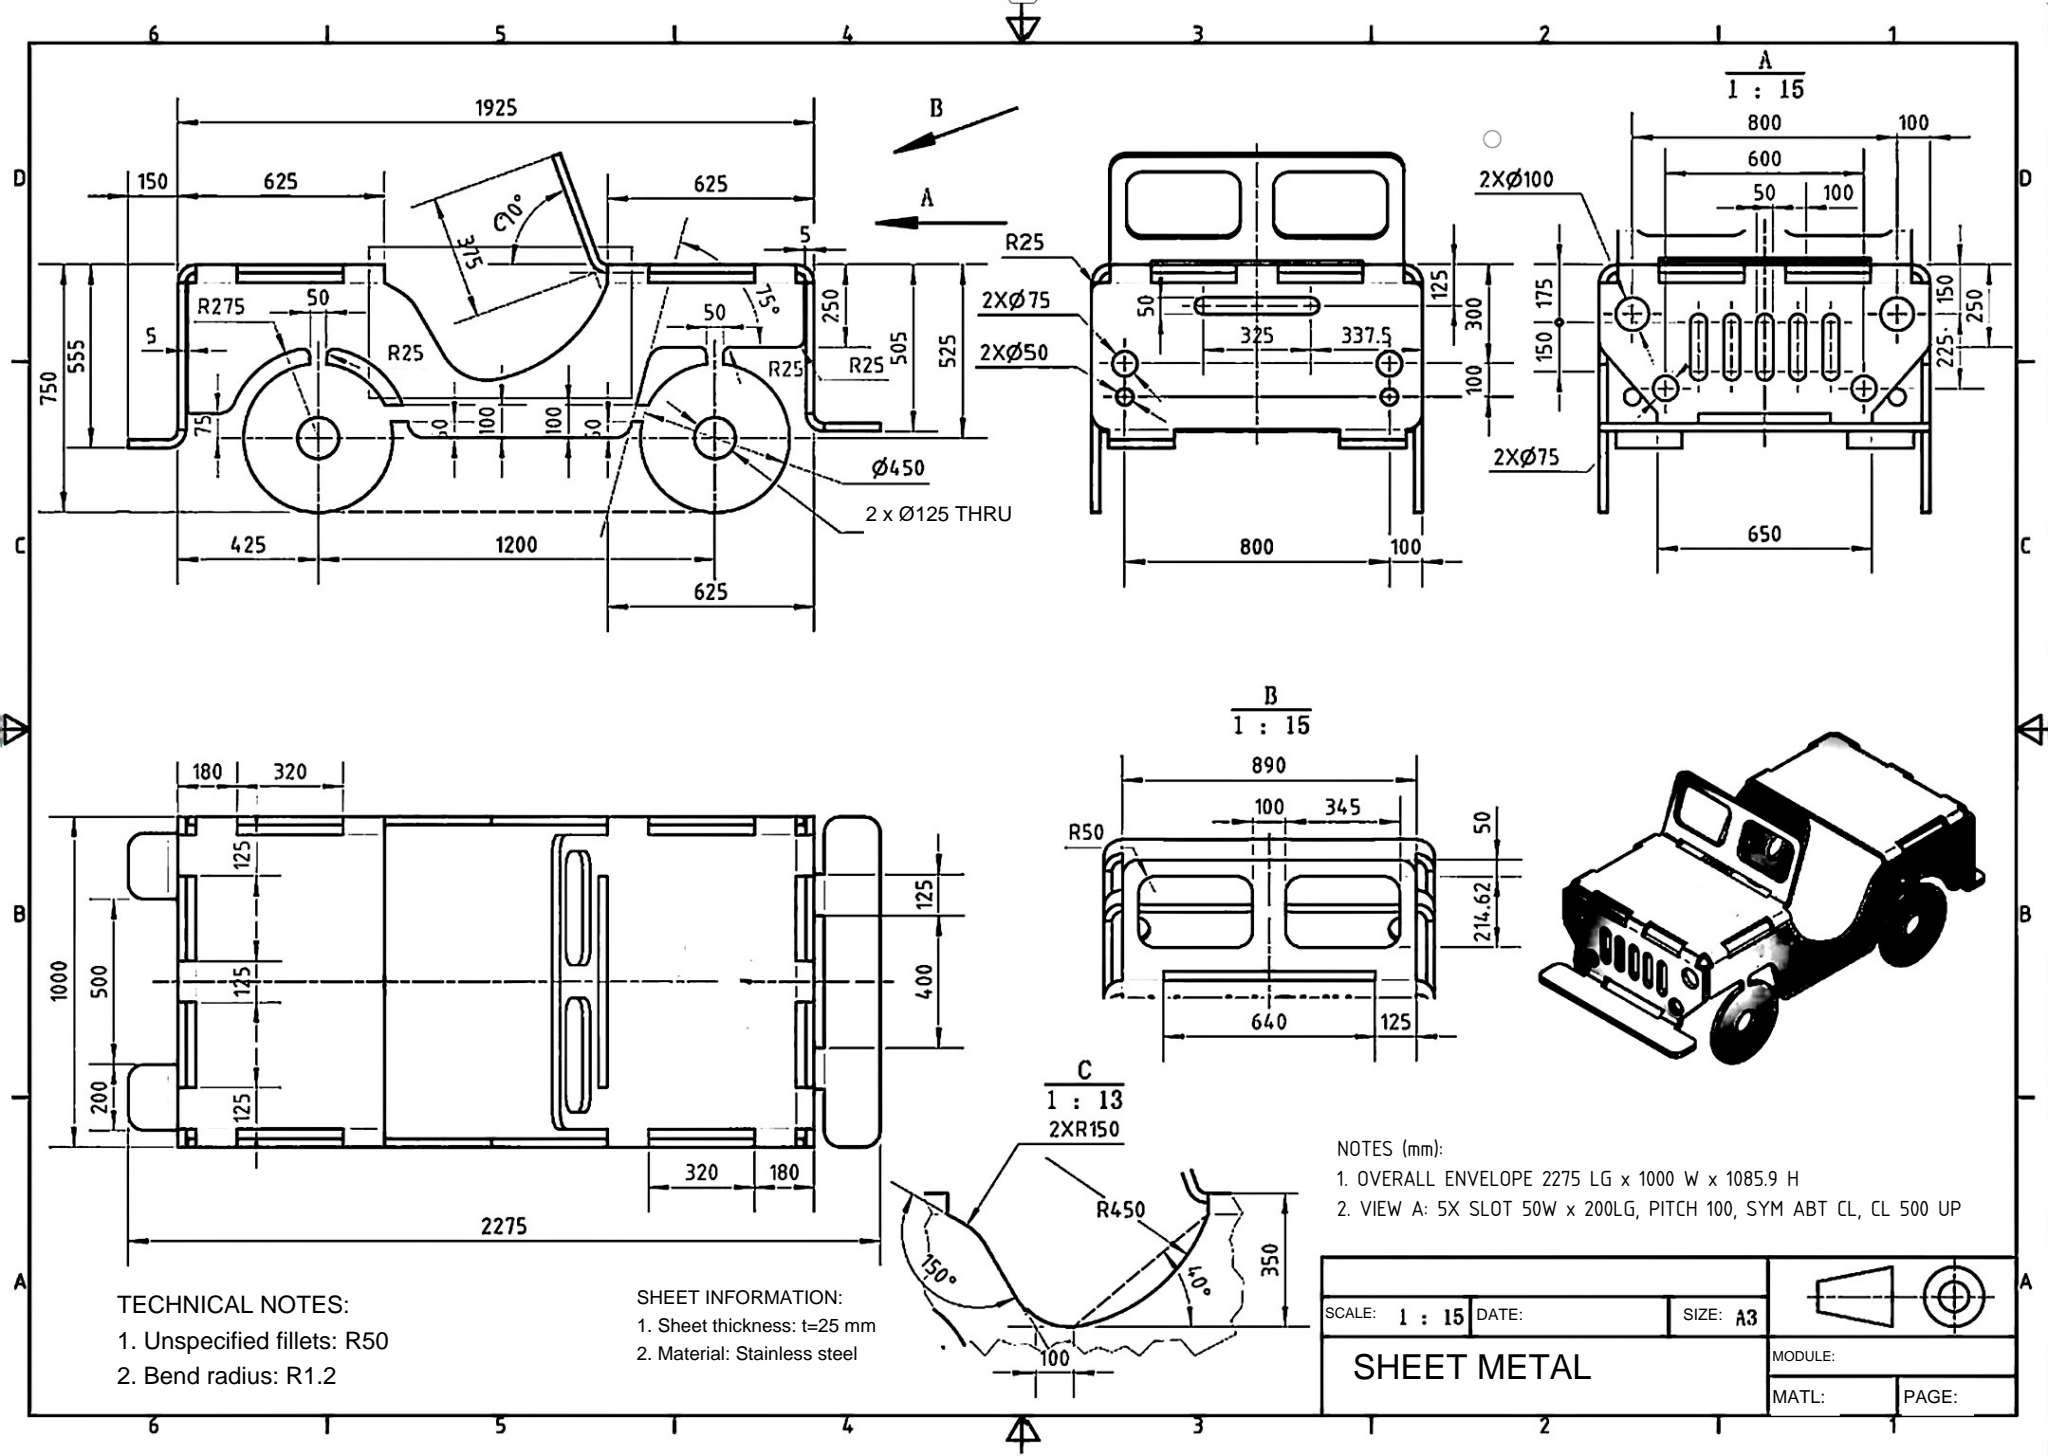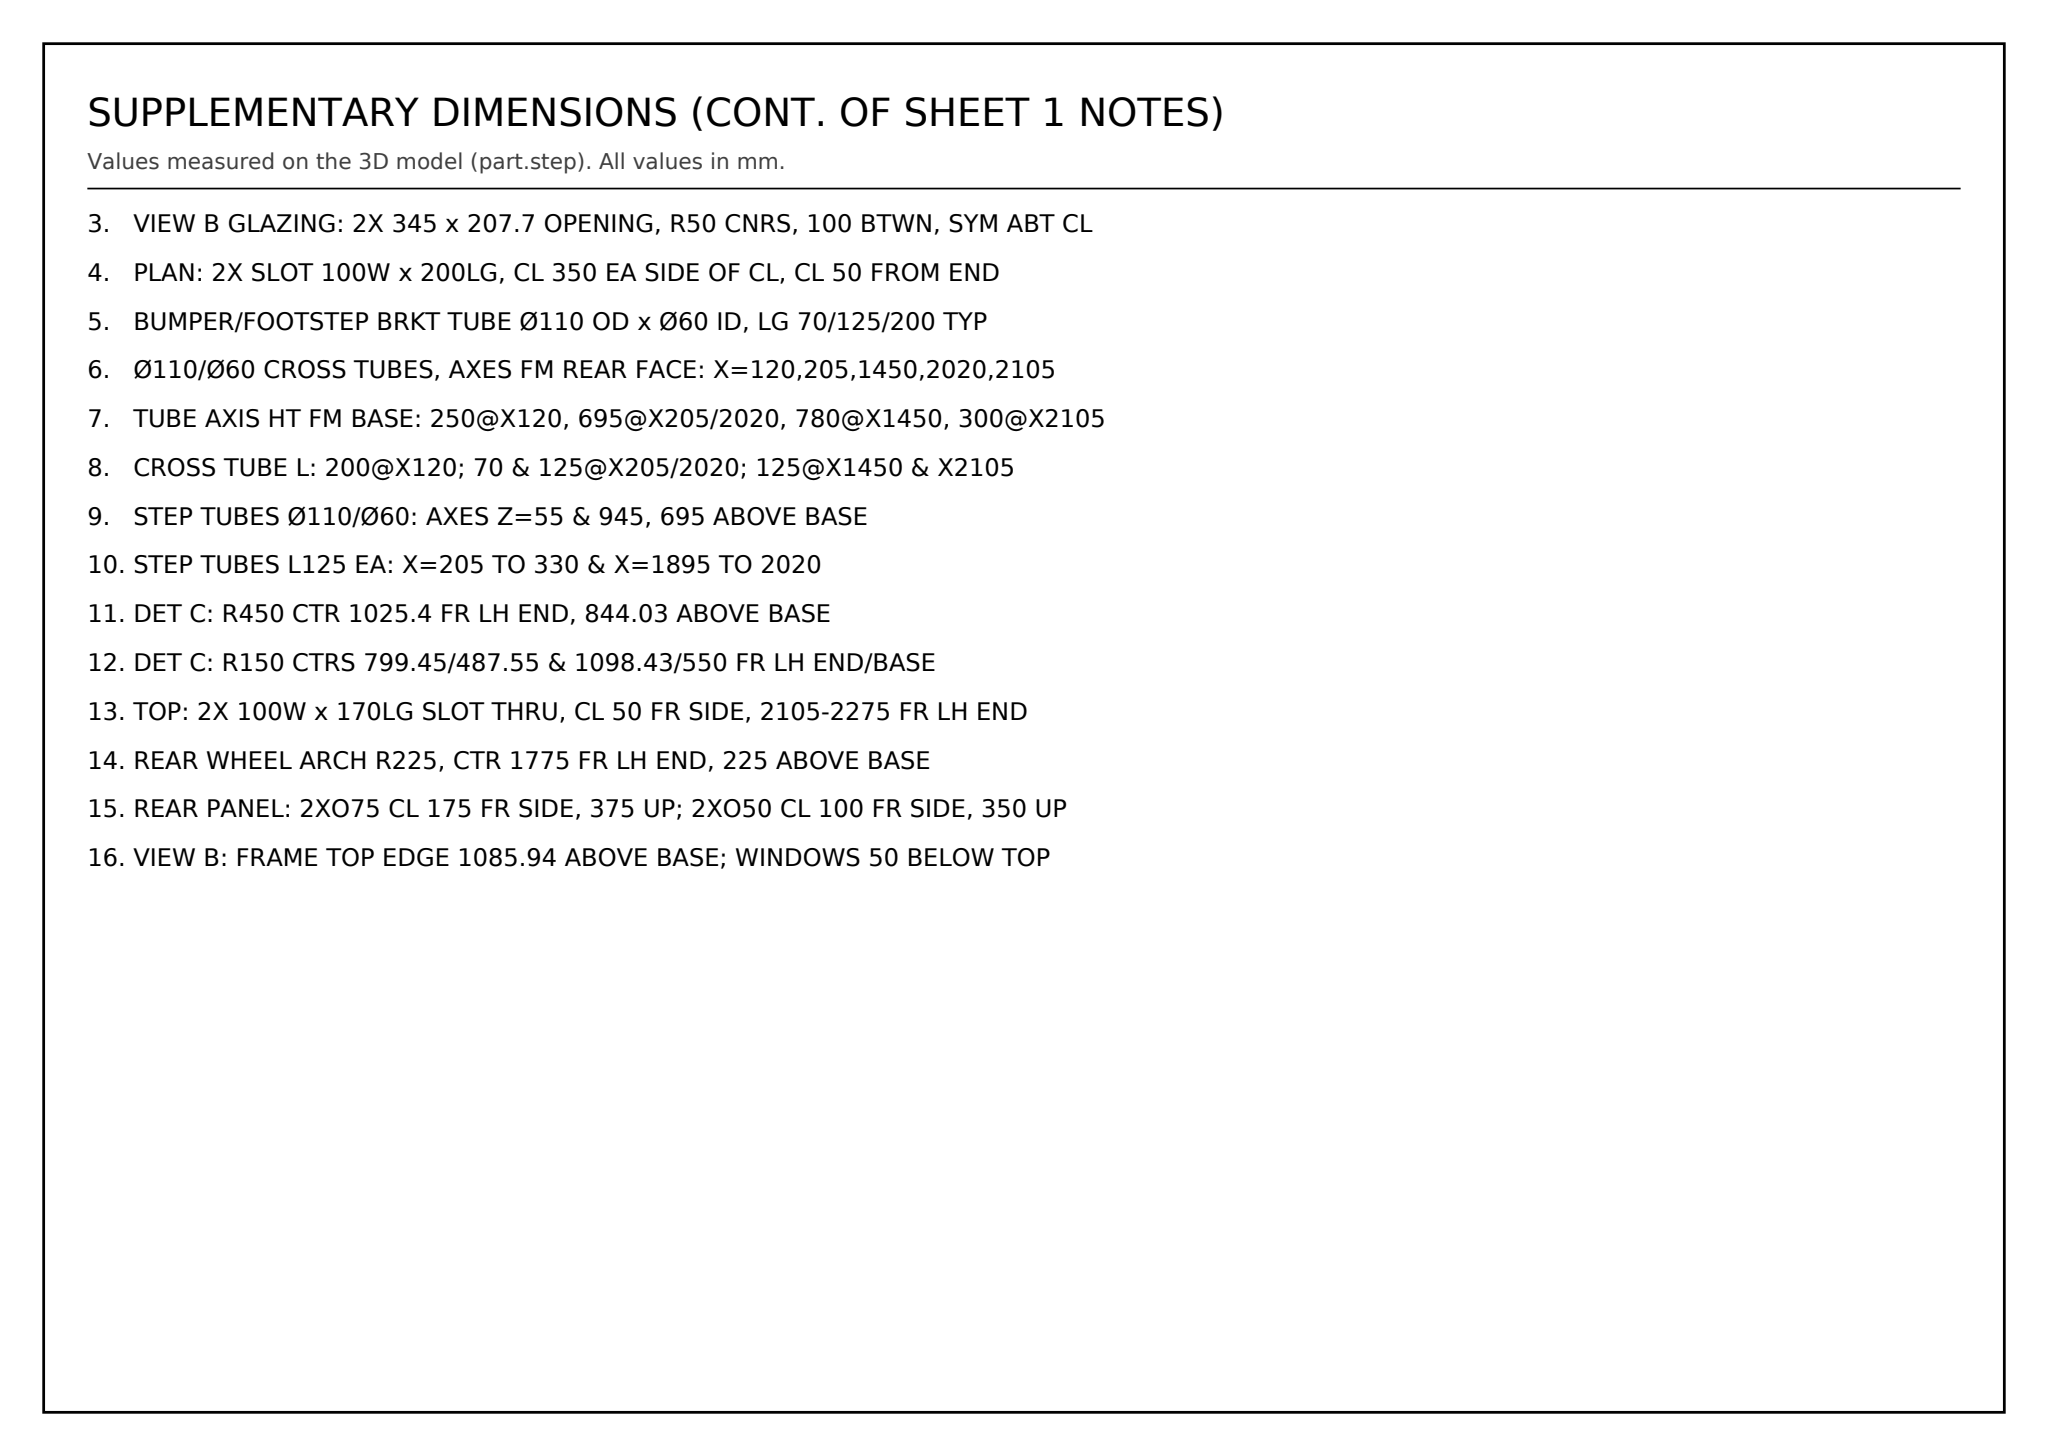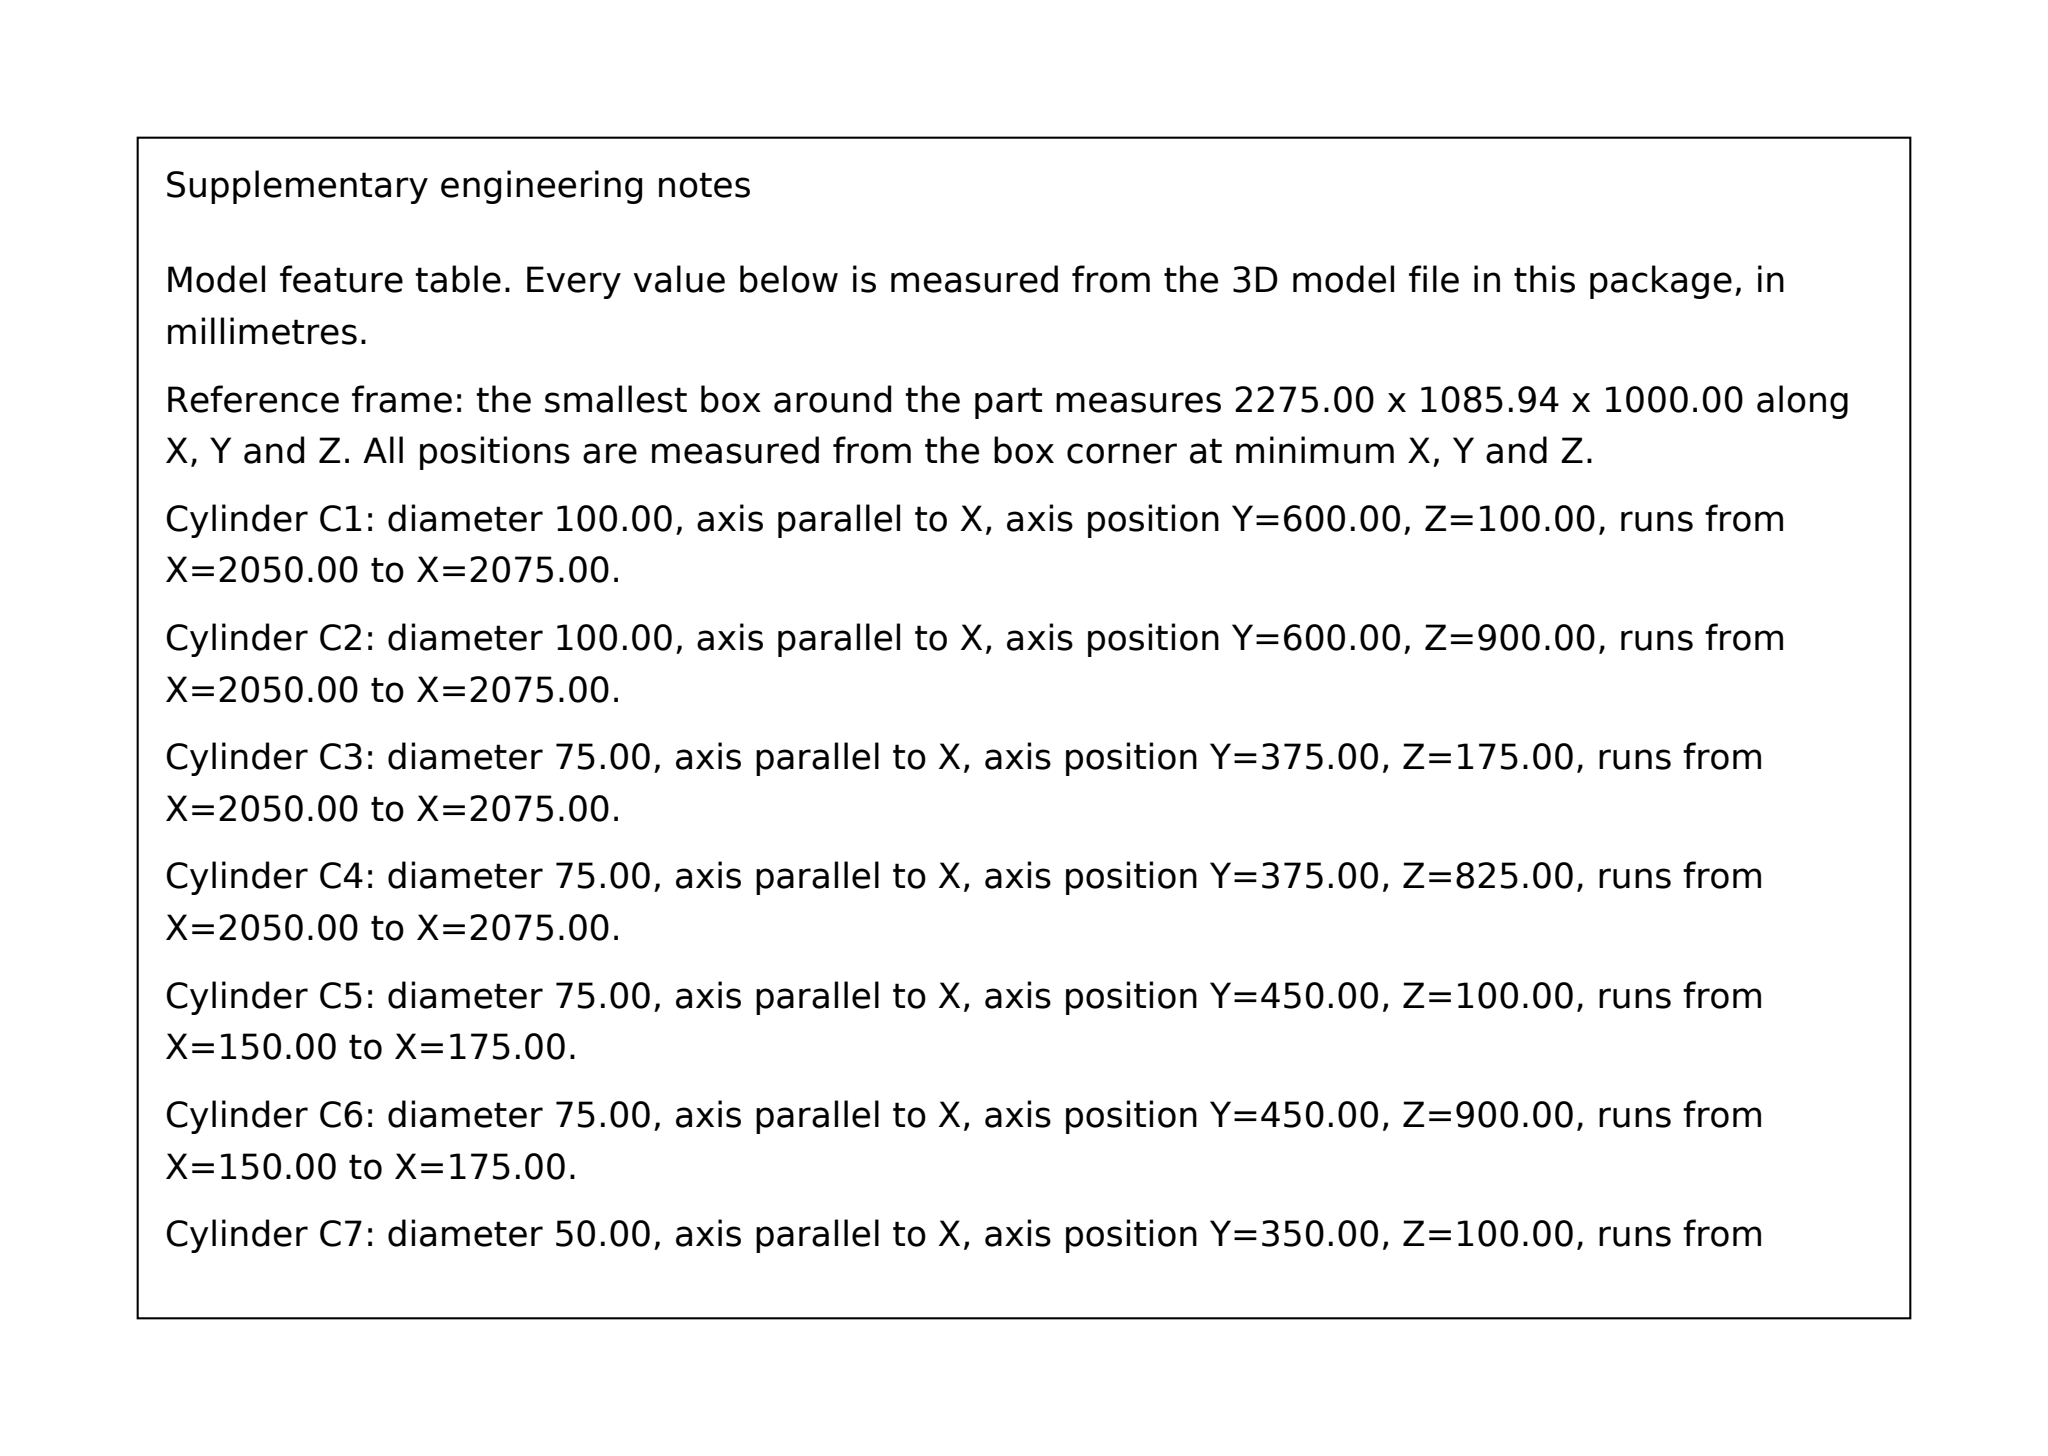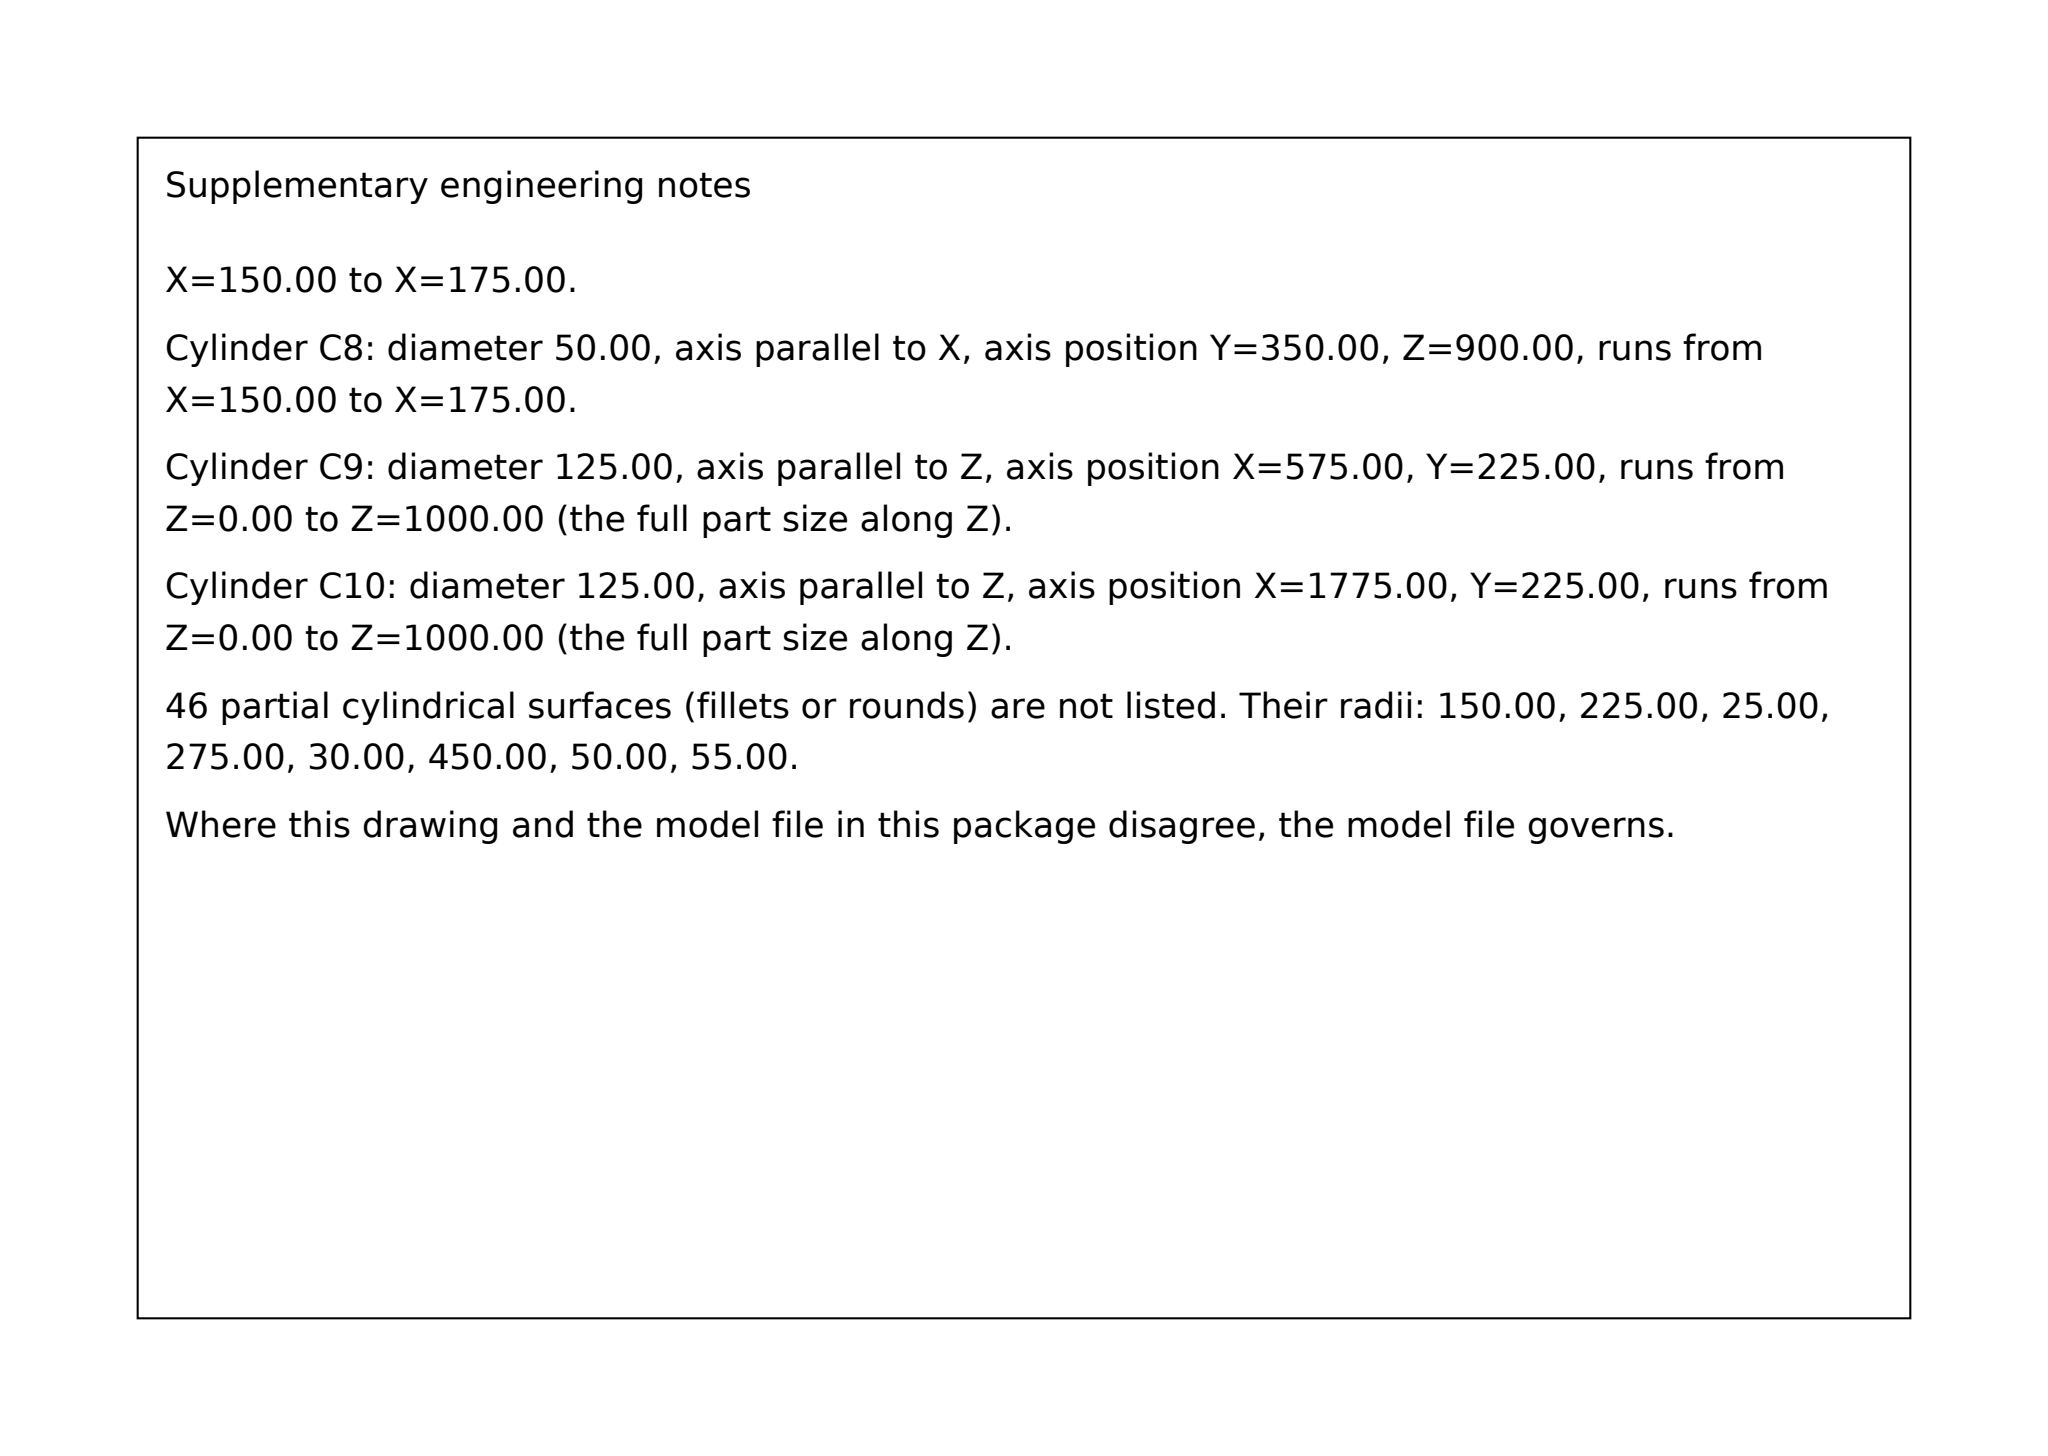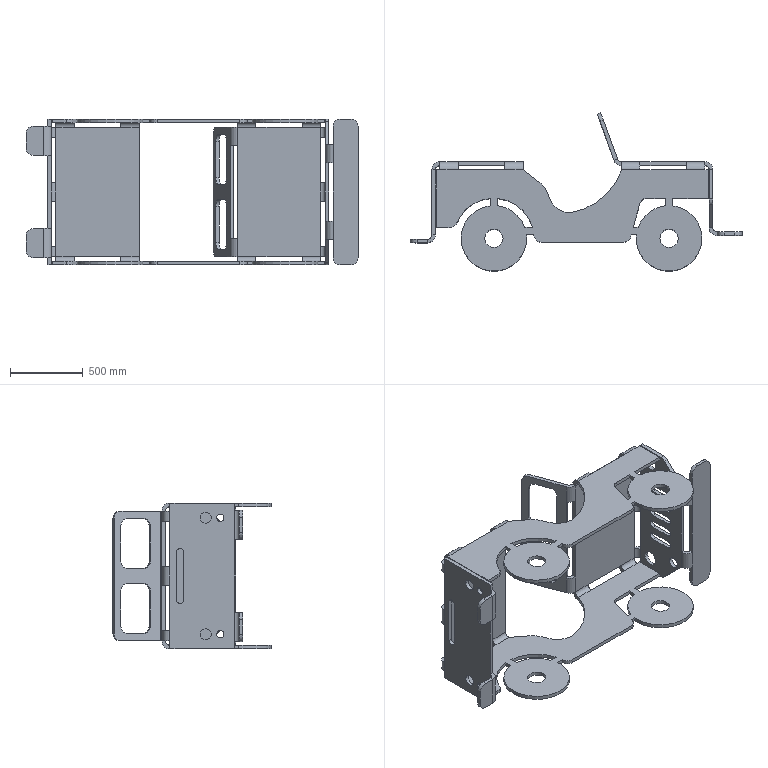Part | SolidWorks | mm | 1 solid | 303 faces | box 2275 x 1085.94 x 1000 mm | volume 96546180 mm3 | plane 166 | cylinder 137 | commonest cylinder face diameters 100 x32 50 x21 110 x20 60 x20 450 x16 75 x8 125 x8 550 x6
Drawing notes:
OVERALL ENVELOPE 2275 LG x 1000 W x 1085.9 H | from the solid: bbox_xyz = [2275.0, 1085.935, 1000.0]
VIEW A: 5X SLOT 50W x 200LG, PITCH 100, SYM ABT CL, CL 500 UP | from the solid: Ø50 x-axis cyls at y=425 & 575, z=300/400/500/600/700, L=25: 50 wide x 200 long slots, 100 pitch, sym about z=500, slot CL y=500 above bbox bottom
VIEW B GLAZING: 2X 345 x 207.7 OPENING, R50 CNRS, 100 BTWN, SYM ABT CL | from the solid: Ø100 x-axis cnr cyls L=40.59 at y=1195.46 & 1303.16, z=155/400 and 600/845 -> 345 x 207.7 openings, R50 cnrs, 100 gap, sym about z=500
PLAN: 2X SLOT 100W x 200LG, CL 350 EA SIDE OF CL, CL 50 FROM END | from the solid: Ø100 y-axis cyls at x=50, z=100 & 200 and z=800 & 900: 100 wide x 200 long slots, CL z=150 & 850 (350 off CL z=500), slot CL x=50 from end face x=0
BUMPER/FOOTSTEP BRKT TUBE Ø110 OD x Ø60 ID, LG 70/125/200 TYP | from the solid: Coaxial Ø60/Ø110 pairs: z-axis at (120,250) L=200, (205,695) L=70 & 125, (1450,780) L=125, (2020,695) L=70 & 125, (2105,300) L=125; x-axis at y=695, z=55 & 945 L=125
Ø110/Ø60 CROSS TUBES, AXES FM REAR FACE: X=120,205,1450,2020,2105 | from the solid: cylinders dia110/60 axis z at x=120,205,1450,2020,2105; bbox x 0-2275
TUBE AXIS HT FM BASE: 250@X120, 695@X205/2020, 780@X1450, 300@X2105 | from the solid: dia110 axis z pos_other y = 250,695,780,695,300 respectively
CROSS TUBE L: 200@X120; 70 & 125@X205/2020; 125@X1450 & X2105 | from the solid: lengths 200,70,125,125,70,125,125 for dia110 z-axis cylinders
STEP TUBES Ø110/Ø60: AXES Z=55 & 945, 695 ABOVE BASE | from the solid: dia110/60 axis x at [y=695,z=55] and [y=695,z=945]
STEP TUBES L125 EA: X=205 TO 330 & X=1895 TO 2020 | from the solid: x-axis tube length 125; axis_planes x=205(4),330(2),1895(2),2020(4)
DET C: R450 CTR 1025.4 FR LH END, 844.03 ABOVE BASE | from the solid: cyl dia 900, axis z, pos (1025.40, 844.03) -> R450 arc centre
DET C: R150 CTRS 799.45/487.55 & 1098.43/550 FR LH END/BASE | from the solid: cyl dia 300, axis z, pos (799.45, 487.55) and (1098.43, 550.0) -> 2XR150 centres
TOP: 2X 100W x 170LG SLOT THRU, CL 50 FR SIDE, 2105-2275 FR LH END | from the solid: dia 100 axis y holes at x=2155 & 2225, z=50 & 950, L=25 -> slot 100W, ends 2105/2275, CL 50 from z0 & z1000
REAR WHEEL ARCH R225, CTR 1775 FR LH END, 225 ABOVE BASE | from the solid: cyl dia 450 axis z at (1775.0, 225.0); front arch same dia at (575.0,225.0) with dia 550 = R275
REAR PANEL: 2XO75 CL 175 FR SIDE, 375 UP; 2XO50 CL 100 FR SIDE, 350 UP | from the solid: dia 75 axis x at y375/z175 & z825; dia 50 axis x at y350/z100 & z900 -> 75 lateral, 25 vert offset
VIEW B: FRAME TOP EDGE 1085.94 ABOVE BASE; WINDOWS 50 BELOW TOP | from the solid: bbox y max = 1085.935 (base y=0); window corner R50 cyls dia 100 give 345 wide openings, 100 apart